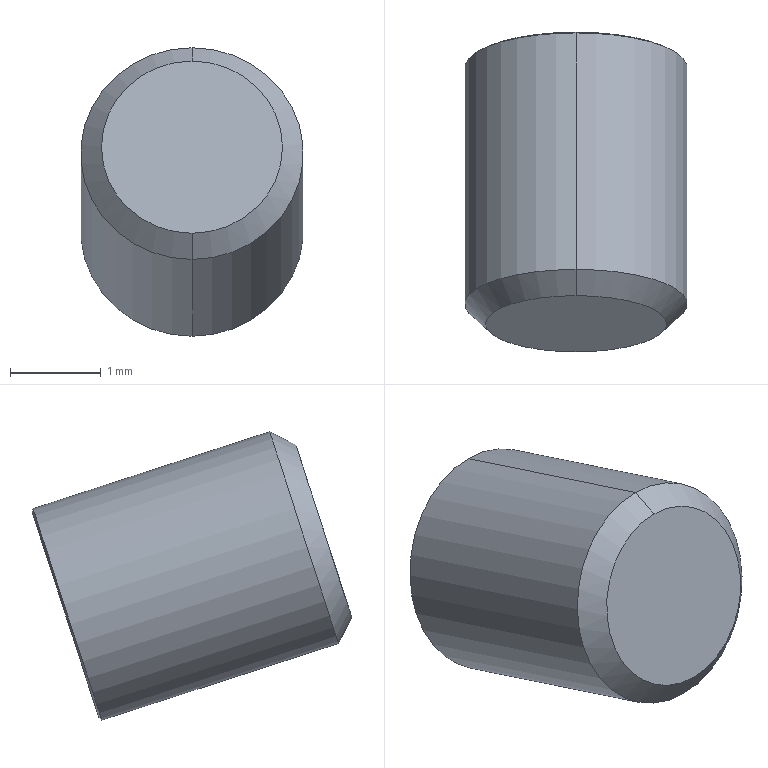Component | SolidWorks | Gewindestift_DIN_913_M3x3-1 | 1 solid | 22 faces | box 2.46 x 3.53 x 3.19 mm | volume 12 mm3 | cone 11 | plane 9 | cylinder 2 | commonest cylinder face diameters 2.459 x2
STEP:
#1=COLOUR_RGB('',0.7922,0.8196,0.9333);
#2=FILL_AREA_STYLE_COLOUR('',#1);
#3=FILL_AREA_STYLE('',(#2));
#4=SURFACE_STYLE_FILL_AREA(#3);
#5=SURFACE_SIDE_STYLE('',(#4));
#6=SURFACE_STYLE_USAGE(.BOTH.,#5);
#7=PRESENTATION_STYLE_ASSIGNMENT((#6));
#8=CARTESIAN_POINT('',(-0.5195,0.1896,-4.016));
#9=VERTEX_POINT('',#8);
#10=CARTESIAN_POINT('',(-0.5195,0.2186,-3.927));
#11=VERTEX_POINT('',#10);
#12=CARTESIAN_POINT('',(-0.5195,0.2041,-3.971));
#13=DIRECTION('',(0.,0.9512,-0.3087));
#14=DIRECTION('',(-0.,-0.3087,-0.9512));
#15=AXIS2_PLACEMENT_3D('',#12,#13,#14);
#16=CIRCLE('',#15,0.04699);
#17=EDGE_CURVE('',#9,#11,#16,.T.);
#18=ORIENTED_EDGE('',*,*,#17,.F.);
#19=CARTESIAN_POINT('',(-0.5195,0.1884,-4.017));
#20=VERTEX_POINT('',#19);
#21=CARTESIAN_POINT('',(-0.5195,0.1896,-4.016));
#22=DIRECTION('',(-0.,-0.7429,-0.6694));
#23=VECTOR('',#22,39.37);
#24=LINE('',#21,#23);
#25=EDGE_CURVE('',#9,#20,#24,.T.);
#26=ORIENTED_EDGE('',*,*,#25,.T.);
#27=CARTESIAN_POINT('',(-0.5195,0.2183,-3.925));
#28=VERTEX_POINT('',#27);
#29=CARTESIAN_POINT('',(-0.5195,0.2033,-3.971));
#30=DIRECTION('',(0.,0.9512,-0.3087));
#31=DIRECTION('',(-0.,0.3087,0.9512));
#32=AXIS2_PLACEMENT_3D('',#29,#30,#31);
#33=CIRCLE('',#32,0.04841);
#34=EDGE_CURVE('',#20,#28,#33,.T.);
#35=ORIENTED_EDGE('',*,*,#34,.T.);
#36=CARTESIAN_POINT('',(-0.5195,0.2186,-3.927));
#37=DIRECTION('',(0.,-0.2082,0.9781));
#38=VECTOR('',#37,39.37);
#39=LINE('',#36,#38);
#40=EDGE_CURVE('',#11,#28,#39,.T.);
#41=ORIENTED_EDGE('',*,*,#40,.F.);
#42=EDGE_LOOP('',(#18,#26,#35,#41));
#43=FACE_OUTER_BOUND('',#42,.T.);
#44=CARTESIAN_POINT('',(-0.5195,0.2041,-3.971));
#45=DIRECTION('',(-0.,-0.9512,0.3087));
#46=DIRECTION('',(0.,0.3087,0.9512));
#47=AXIS2_PLACEMENT_3D('',#44,#45,#46);
#48=CONICAL_SURFACE('',#47,0.04699,1.047);
#49=ADVANCED_FACE('',(#43),#48,.T.);
#50=CARTESIAN_POINT('',(-0.5195,0.08541,-3.984));
#51=VERTEX_POINT('',#50);
#52=CARTESIAN_POINT('',(-0.5195,0.1153,-3.892));
#53=VERTEX_POINT('',#52);
#54=CARTESIAN_POINT('',(-0.5195,0.1004,-3.938));
#55=DIRECTION('',(0.,0.9512,-0.3087));
#56=DIRECTION('',(-0.,-0.3087,-0.9512));
#57=AXIS2_PLACEMENT_3D('',#54,#55,#56);
#58=CIRCLE('',#57,0.04841);
#59=EDGE_CURVE('',#51,#53,#58,.T.);
#60=ORIENTED_EDGE('',*,*,#59,.T.);
#61=CARTESIAN_POINT('',(-0.5195,0.2003,-3.919));
#62=DIRECTION('',(0.,0.9512,-0.3087));
#63=VECTOR('',#62,39.37);
#64=LINE('',#61,#63);
#65=EDGE_CURVE('',#53,#28,#64,.T.);
#66=ORIENTED_EDGE('',*,*,#65,.T.);
#67=ORIENTED_EDGE('',*,*,#34,.F.);
#68=CARTESIAN_POINT('',(-0.5195,0.1704,-4.011));
#69=DIRECTION('',(0.,0.9512,-0.3087));
#70=VECTOR('',#69,39.37);
#71=LINE('',#68,#70);
#72=EDGE_CURVE('',#51,#20,#71,.T.);
#73=ORIENTED_EDGE('',*,*,#72,.F.);
#74=EDGE_LOOP('',(#60,#66,#67,#73));
#75=FACE_OUTER_BOUND('',#74,.T.);
#76=CARTESIAN_POINT('',(-0.5195,0.1854,-3.965));
#77=DIRECTION('',(0.,0.9512,-0.3087));
#78=DIRECTION('',(-0.,-0.3087,-0.9512));
#79=AXIS2_PLACEMENT_3D('',#76,#77,#78);
#80=CYLINDRICAL_SURFACE('',#79,0.04841);
#81=ADVANCED_FACE('',(#75),#80,.T.);
#82=CARTESIAN_POINT('',(-0.5195,0.07961,-3.972));
#83=VERTEX_POINT('',#82);
#84=CARTESIAN_POINT('',(-0.5195,0.1039,-3.897));
#85=VERTEX_POINT('',#84);
#86=CARTESIAN_POINT('',(-0.5195,0.09176,-3.935));
#87=DIRECTION('',(0.,0.9512,-0.3087));
#88=DIRECTION('',(-0.,-0.3087,-0.9512));
#89=AXIS2_PLACEMENT_3D('',#86,#87,#88);
#90=CIRCLE('',#89,0.03937);
#91=EDGE_CURVE('',#83,#85,#90,.T.);
#92=ORIENTED_EDGE('',*,*,#91,.T.);
#93=CARTESIAN_POINT('',(-0.5195,0.1287,-3.885));
#94=DIRECTION('',(0.,0.8909,0.4543));
#95=VECTOR('',#94,39.37);
#96=LINE('',#93,#95);
#97=EDGE_CURVE('',#85,#53,#96,.T.);
#98=ORIENTED_EDGE('',*,*,#97,.T.);
#99=ORIENTED_EDGE('',*,*,#59,.F.);
#100=CARTESIAN_POINT('',(-0.5195,0.09225,-3.997));
#101=DIRECTION('',(0.,0.4543,-0.8909));
#102=VECTOR('',#101,39.37);
#103=LINE('',#100,#102);
#104=EDGE_CURVE('',#83,#51,#103,.T.);
#105=ORIENTED_EDGE('',*,*,#104,.F.);
#106=EDGE_LOOP('',(#92,#98,#99,#105));
#107=FACE_OUTER_BOUND('',#106,.T.);
#108=CARTESIAN_POINT('',(-0.5195,0.1105,-3.941));
#109=DIRECTION('',(0.,0.9512,-0.3087));
#110=DIRECTION('',(-0.,-0.3087,-0.9512));
#111=AXIS2_PLACEMENT_3D('',#108,#109,#110);
#112=CONICAL_SURFACE('',#111,0.05906,0.7854);
#113=ADVANCED_FACE('',(#107),#112,.T.);
#114=CARTESIAN_POINT('',(-0.5365,0.195,-3.999));
#115=VERTEX_POINT('',#114);
#116=CARTESIAN_POINT('',(-0.5195,0.1925,-3.999));
#117=VERTEX_POINT('',#116);
#118=CARTESIAN_POINT('',(-0.5365,0.195,-3.999));
#119=CARTESIAN_POINT('',(-0.531,0.1935,-3.999));
#120=CARTESIAN_POINT('',(-0.5252,0.1925,-3.999));
#121=CARTESIAN_POINT('',(-0.5195,0.1925,-3.999));
#122=B_SPLINE_CURVE_WITH_KNOTS('',3,(#118,#119,#120,#121),.UNSPECIFIED.,.F.,.F.,(4,4),(0.002319,0.002758),.UNSPECIFIED.);
#123=EDGE_CURVE('',#115,#117,#122,.T.);
#124=ORIENTED_EDGE('',*,*,#123,.T.);
#125=CARTESIAN_POINT('',(-0.5195,0.1936,-4.004));
#126=VERTEX_POINT('',#125);
#127=CARTESIAN_POINT('',(-0.5195,0.1854,-3.965));
#128=DIRECTION('',(-0.,0.2082,-0.9781));
#129=VECTOR('',#128,39.37);
#130=LINE('',#127,#129);
#131=EDGE_CURVE('',#117,#126,#130,.T.);
#132=ORIENTED_EDGE('',*,*,#131,.T.);
#133=CARTESIAN_POINT('',(-0.5195,0.2041,-3.971));
#134=DIRECTION('',(0.,0.9512,-0.3087));
#135=DIRECTION('',(-0.,-0.3087,-0.9512));
#136=AXIS2_PLACEMENT_3D('',#133,#134,#135);
#137=CIRCLE('',#136,0.0341);
#138=EDGE_CURVE('',#126,#115,#137,.T.);
#139=ORIENTED_EDGE('',*,*,#138,.T.);
#140=EDGE_LOOP('',(#124,#132,#139));
#141=FACE_OUTER_BOUND('',#140,.T.);
#142=CARTESIAN_POINT('',(-0.5195,37.633,-16.119));
#143=DIRECTION('',(0.,0.9512,-0.3087));
#144=DIRECTION('',(-0.,-0.3087,-0.9512));
#145=AXIS2_PLACEMENT_3D('',#142,#143,#144);
#146=CONICAL_SURFACE('',#145,68.191,1.047);
#147=ADVANCED_FACE('',(#141),#146,.F.);
#148=CARTESIAN_POINT('',(-0.5536,0.2041,-3.971));
#149=VERTEX_POINT('',#148);
#150=CARTESIAN_POINT('',(-0.5365,0.2132,-3.943));
#151=VERTEX_POINT('',#150);
#152=CARTESIAN_POINT('',(-0.5195,0.2041,-3.971));
#153=DIRECTION('',(0.,0.9512,-0.3087));
#154=DIRECTION('',(-0.,-0.3087,-0.9512));
#155=AXIS2_PLACEMENT_3D('',#152,#153,#154);
#156=CIRCLE('',#155,0.0341);
#157=EDGE_CURVE('',#149,#151,#156,.T.);
#158=ORIENTED_EDGE('',*,*,#157,.T.);
#159=CARTESIAN_POINT('',(-0.5365,0.2132,-3.943));
#160=CARTESIAN_POINT('',(-0.5393,0.2102,-3.947));
#161=CARTESIAN_POINT('',(-0.5421,0.2077,-3.952));
#162=CARTESIAN_POINT('',(-0.5479,0.2046,-3.961));
#163=CARTESIAN_POINT('',(-0.5508,0.2041,-3.966));
#164=CARTESIAN_POINT('',(-0.5536,0.2041,-3.971));
#165=B_SPLINE_CURVE_WITH_KNOTS('',3,(#159,#160,#161,#162,#163,#164),.UNSPECIFIED.,.F.,.F.,(4,2,4),(0.00000024,0.0004376,0.0008749),.UNSPECIFIED.);
#166=EDGE_CURVE('',#151,#149,#165,.T.);
#167=ORIENTED_EDGE('',*,*,#166,.T.);
#168=EDGE_LOOP('',(#158,#167));
#169=FACE_OUTER_BOUND('',#168,.T.);
#170=CARTESIAN_POINT('',(-0.5195,37.633,-16.119));
#171=DIRECTION('',(0.,0.9512,-0.3087));
#172=DIRECTION('',(-0.,-0.3087,-0.9512));
#173=AXIS2_PLACEMENT_3D('',#170,#171,#172);
#174=CONICAL_SURFACE('',#173,68.191,1.047);
#175=ADVANCED_FACE('',(#169),#174,.F.);
#176=CARTESIAN_POINT('',(-0.5195,0.2041,-3.971));
#177=DIRECTION('',(0.,0.9512,-0.3087));
#178=DIRECTION('',(-0.,-0.3087,-0.9512));
#179=AXIS2_PLACEMENT_3D('',#176,#177,#178);
#180=CIRCLE('',#179,0.0341);
#181=EDGE_CURVE('',#115,#149,#180,.T.);
#182=ORIENTED_EDGE('',*,*,#181,.T.);
#183=CARTESIAN_POINT('',(-0.5536,0.2041,-3.971));
#184=CARTESIAN_POINT('',(-0.5508,0.2011,-3.975));
#185=CARTESIAN_POINT('',(-0.548,0.1986,-3.98));
#186=CARTESIAN_POINT('',(-0.5422,0.1955,-3.989));
#187=CARTESIAN_POINT('',(-0.5393,0.1949,-3.994));
#188=CARTESIAN_POINT('',(-0.5365,0.195,-3.999));
#189=B_SPLINE_CURVE_WITH_KNOTS('',3,(#183,#184,#185,#186,#187,#188),.UNSPECIFIED.,.F.,.F.,(4,2,4),(0.00000024,0.0004376,0.0008749),.UNSPECIFIED.);
#190=EDGE_CURVE('',#149,#115,#189,.T.);
#191=ORIENTED_EDGE('',*,*,#190,.T.);
#192=EDGE_LOOP('',(#182,#191));
#193=FACE_OUTER_BOUND('',#192,.T.);
#194=CARTESIAN_POINT('',(-0.5195,37.633,-16.119));
#195=DIRECTION('',(0.,0.9512,-0.3087));
#196=DIRECTION('',(-0.,-0.3087,-0.9512));
#197=AXIS2_PLACEMENT_3D('',#194,#195,#196);
#198=CONICAL_SURFACE('',#197,68.191,1.047);
#199=ADVANCED_FACE('',(#193),#198,.F.);
#200=ORIENTED_EDGE('',*,*,#131,.F.);
#201=CARTESIAN_POINT('',(-0.5024,0.195,-3.999));
#202=VERTEX_POINT('',#201);
#203=CARTESIAN_POINT('',(-0.5195,0.1925,-3.999));
#204=CARTESIAN_POINT('',(-0.5137,0.1925,-3.999));
#205=CARTESIAN_POINT('',(-0.508,0.1935,-3.999));
#206=CARTESIAN_POINT('',(-0.5024,0.195,-3.999));
#207=B_SPLINE_CURVE_WITH_KNOTS('',3,(#203,#204,#205,#206),.UNSPECIFIED.,.F.,.F.,(4,4),(0.002758,0.003196),.UNSPECIFIED.);
#208=EDGE_CURVE('',#117,#202,#207,.T.);
#209=ORIENTED_EDGE('',*,*,#208,.T.);
#210=CARTESIAN_POINT('',(-0.5195,0.2041,-3.971));
#211=DIRECTION('',(0.,0.9512,-0.3087));
#212=DIRECTION('',(-0.,-0.3087,-0.9512));
#213=AXIS2_PLACEMENT_3D('',#210,#211,#212);
#214=CIRCLE('',#213,0.0341);
#215=EDGE_CURVE('',#202,#126,#214,.T.);
#216=ORIENTED_EDGE('',*,*,#215,.T.);
#217=EDGE_LOOP('',(#200,#209,#216));
#218=FACE_OUTER_BOUND('',#217,.T.);
#219=CARTESIAN_POINT('',(-0.5195,37.633,-16.119));
#220=DIRECTION('',(0.,0.9512,-0.3087));
#221=DIRECTION('',(-0.,-0.3087,-0.9512));
#222=AXIS2_PLACEMENT_3D('',#219,#220,#221);
#223=CONICAL_SURFACE('',#222,68.191,1.047);
#224=ADVANCED_FACE('',(#218),#223,.F.);
#225=CARTESIAN_POINT('',(-0.4854,0.2041,-3.971));
#226=VERTEX_POINT('',#225);
#227=CARTESIAN_POINT('',(-0.5195,0.2041,-3.971));
#228=DIRECTION('',(0.,0.9512,-0.3087));
#229=DIRECTION('',(-0.,-0.3087,-0.9512));
#230=AXIS2_PLACEMENT_3D('',#227,#228,#229);
#231=CIRCLE('',#230,0.0341);
#232=EDGE_CURVE('',#226,#202,#231,.T.);
#233=ORIENTED_EDGE('',*,*,#232,.T.);
#234=CARTESIAN_POINT('',(-0.5024,0.195,-3.999));
#235=CARTESIAN_POINT('',(-0.4996,0.1949,-3.994));
#236=CARTESIAN_POINT('',(-0.4968,0.1955,-3.989));
#237=CARTESIAN_POINT('',(-0.491,0.1986,-3.98));
#238=CARTESIAN_POINT('',(-0.4882,0.2011,-3.975));
#239=CARTESIAN_POINT('',(-0.4854,0.2041,-3.971));
#240=B_SPLINE_CURVE_WITH_KNOTS('',3,(#234,#235,#236,#237,#238,#239),.UNSPECIFIED.,.F.,.F.,(4,2,4),(0.00000024,0.0004376,0.0008749),.UNSPECIFIED.);
#241=EDGE_CURVE('',#202,#226,#240,.T.);
#242=ORIENTED_EDGE('',*,*,#241,.T.);
#243=EDGE_LOOP('',(#233,#242));
#244=FACE_OUTER_BOUND('',#243,.T.);
#245=CARTESIAN_POINT('',(-0.5195,37.633,-16.119));
#246=DIRECTION('',(0.,0.9512,-0.3087));
#247=DIRECTION('',(-0.,-0.3087,-0.9512));
#248=AXIS2_PLACEMENT_3D('',#245,#246,#247);
#249=CONICAL_SURFACE('',#248,68.191,1.047);
#250=ADVANCED_FACE('',(#244),#249,.F.);
#251=CARTESIAN_POINT('',(-0.5024,0.2132,-3.943));
#252=VERTEX_POINT('',#251);
#253=CARTESIAN_POINT('',(-0.5195,0.2041,-3.971));
#254=DIRECTION('',(0.,0.9512,-0.3087));
#255=DIRECTION('',(-0.,-0.3087,-0.9512));
#256=AXIS2_PLACEMENT_3D('',#253,#254,#255);
#257=CIRCLE('',#256,0.0341);
#258=EDGE_CURVE('',#252,#226,#257,.T.);
#259=ORIENTED_EDGE('',*,*,#258,.T.);
#260=CARTESIAN_POINT('',(-0.4854,0.2041,-3.971));
#261=CARTESIAN_POINT('',(-0.4882,0.2041,-3.966));
#262=CARTESIAN_POINT('',(-0.491,0.2046,-3.961));
#263=CARTESIAN_POINT('',(-0.4968,0.2077,-3.952));
#264=CARTESIAN_POINT('',(-0.4996,0.2102,-3.947));
#265=CARTESIAN_POINT('',(-0.5024,0.2132,-3.943));
#266=B_SPLINE_CURVE_WITH_KNOTS('',3,(#260,#261,#262,#263,#264,#265),.UNSPECIFIED.,.F.,.F.,(4,2,4),(0.00000024,0.0004376,0.0008749),.UNSPECIFIED.);
#267=EDGE_CURVE('',#226,#252,#266,.T.);
#268=ORIENTED_EDGE('',*,*,#267,.T.);
#269=EDGE_LOOP('',(#259,#268));
#270=FACE_OUTER_BOUND('',#269,.T.);
#271=CARTESIAN_POINT('',(-0.5195,37.633,-16.119));
#272=DIRECTION('',(0.,0.9512,-0.3087));
#273=DIRECTION('',(-0.,-0.3087,-0.9512));
#274=AXIS2_PLACEMENT_3D('',#271,#272,#273);
#275=CONICAL_SURFACE('',#274,68.191,1.047);
#276=ADVANCED_FACE('',(#270),#275,.F.);
#277=CARTESIAN_POINT('',(-0.5195,0.2041,-3.971));
#278=DIRECTION('',(0.,0.9512,-0.3087));
#279=DIRECTION('',(-0.,-0.3087,-0.9512));
#280=AXIS2_PLACEMENT_3D('',#277,#278,#279);
#281=CIRCLE('',#280,0.0341);
#282=EDGE_CURVE('',#151,#252,#281,.T.);
#283=ORIENTED_EDGE('',*,*,#282,.T.);
#284=CARTESIAN_POINT('',(-0.5024,0.2132,-3.943));
#285=CARTESIAN_POINT('',(-0.508,0.2117,-3.943));
#286=CARTESIAN_POINT('',(-0.5137,0.2107,-3.942));
#287=CARTESIAN_POINT('',(-0.5252,0.2107,-3.942));
#288=CARTESIAN_POINT('',(-0.531,0.2117,-3.943));
#289=CARTESIAN_POINT('',(-0.5365,0.2132,-3.943));
#290=B_SPLINE_CURVE_WITH_KNOTS('',3,(#284,#285,#286,#287,#288,#289),.UNSPECIFIED.,.F.,.F.,(4,2,4),(0.0007425,0.00118,0.001618),.UNSPECIFIED.);
#291=EDGE_CURVE('',#252,#151,#290,.T.);
#292=ORIENTED_EDGE('',*,*,#291,.T.);
#293=EDGE_LOOP('',(#283,#292));
#294=FACE_OUTER_BOUND('',#293,.T.);
#295=CARTESIAN_POINT('',(-0.5195,37.633,-16.119));
#296=DIRECTION('',(0.,0.9512,-0.3087));
#297=DIRECTION('',(-0.,-0.3087,-0.9512));
#298=AXIS2_PLACEMENT_3D('',#295,#296,#297);
#299=CONICAL_SURFACE('',#298,68.191,1.047);
#300=ADVANCED_FACE('',(#294),#299,.F.);
#301=ORIENTED_EDGE('',*,*,#91,.F.);
#302=CARTESIAN_POINT('',(-0.5195,0.09176,-3.935));
#303=DIRECTION('',(0.,0.9512,-0.3087));
#304=DIRECTION('',(-0.,-0.3087,-0.9512));
#305=AXIS2_PLACEMENT_3D('',#302,#303,#304);
#306=CIRCLE('',#305,0.03937);
#307=EDGE_CURVE('',#85,#83,#306,.T.);
#308=ORIENTED_EDGE('',*,*,#307,.F.);
#309=EDGE_LOOP('',(#301,#308));
#310=FACE_OUTER_BOUND('',#309,.T.);
#311=CARTESIAN_POINT('',(-0.5195,0.09176,-3.935));
#312=DIRECTION('',(-0.,-0.9512,0.3087));
#313=DIRECTION('',(0.,0.3087,0.9512));
#314=AXIS2_PLACEMENT_3D('',#311,#312,#313);
#315=PLANE('',#314);
#316=ADVANCED_FACE('',(#310),#315,.T.);
#317=ORIENTED_EDGE('',*,*,#97,.F.);
#318=ORIENTED_EDGE('',*,*,#307,.T.);
#319=ORIENTED_EDGE('',*,*,#104,.T.);
#320=CARTESIAN_POINT('',(-0.5195,0.1004,-3.938));
#321=DIRECTION('',(0.,0.9512,-0.3087));
#322=DIRECTION('',(-0.,-0.3087,-0.9512));
#323=AXIS2_PLACEMENT_3D('',#320,#321,#322);
#324=CIRCLE('',#323,0.04841);
#325=EDGE_CURVE('',#53,#51,#324,.T.);
#326=ORIENTED_EDGE('',*,*,#325,.F.);
#327=EDGE_LOOP('',(#317,#318,#319,#326));
#328=FACE_OUTER_BOUND('',#327,.T.);
#329=CARTESIAN_POINT('',(-0.5195,0.1105,-3.941));
#330=DIRECTION('',(0.,0.9512,-0.3087));
#331=DIRECTION('',(-0.,-0.3087,-0.9512));
#332=AXIS2_PLACEMENT_3D('',#329,#330,#331);
#333=CONICAL_SURFACE('',#332,0.05906,0.7854);
#334=ADVANCED_FACE('',(#328),#333,.T.);
#335=ORIENTED_EDGE('',*,*,#65,.F.);
#336=ORIENTED_EDGE('',*,*,#325,.T.);
#337=ORIENTED_EDGE('',*,*,#72,.T.);
#338=CARTESIAN_POINT('',(-0.5195,0.2033,-3.971));
#339=DIRECTION('',(0.,0.9512,-0.3087));
#340=DIRECTION('',(0.,0.3087,0.9512));
#341=AXIS2_PLACEMENT_3D('',#338,#339,#340);
#342=CIRCLE('',#341,0.04841);
#343=EDGE_CURVE('',#28,#20,#342,.T.);
#344=ORIENTED_EDGE('',*,*,#343,.F.);
#345=EDGE_LOOP('',(#335,#336,#337,#344));
#346=FACE_OUTER_BOUND('',#345,.T.);
#347=CARTESIAN_POINT('',(-0.5195,0.1854,-3.965));
#348=DIRECTION('',(0.,0.9512,-0.3087));
#349=DIRECTION('',(-0.,-0.3087,-0.9512));
#350=AXIS2_PLACEMENT_3D('',#347,#348,#349);
#351=CYLINDRICAL_SURFACE('',#350,0.04841);
#352=ADVANCED_FACE('',(#346),#351,.T.);
#353=ORIENTED_EDGE('',*,*,#25,.F.);
#354=CARTESIAN_POINT('',(-0.5195,0.2041,-3.971));
#355=DIRECTION('',(0.,0.9512,-0.3087));
#356=DIRECTION('',(-0.,-0.3087,-0.9512));
#357=AXIS2_PLACEMENT_3D('',#354,#355,#356);
#358=CIRCLE('',#357,0.04699);
#359=EDGE_CURVE('',#11,#9,#358,.T.);
#360=ORIENTED_EDGE('',*,*,#359,.F.);
#361=ORIENTED_EDGE('',*,*,#40,.T.);
#362=ORIENTED_EDGE('',*,*,#343,.T.);
#363=EDGE_LOOP('',(#353,#360,#361,#362));
#364=FACE_OUTER_BOUND('',#363,.T.);
#365=CARTESIAN_POINT('',(-0.5195,0.2041,-3.971));
#366=DIRECTION('',(-0.,-0.9512,0.3087));
#367=DIRECTION('',(0.,0.3087,0.9512));
#368=AXIS2_PLACEMENT_3D('',#365,#366,#367);
#369=CONICAL_SURFACE('',#368,0.04699,1.047);
#370=ADVANCED_FACE('',(#364),#369,.T.);
#371=ORIENTED_EDGE('',*,*,#359,.T.);
#372=ORIENTED_EDGE('',*,*,#17,.T.);
#373=EDGE_LOOP('',(#371,#372));
#374=FACE_OUTER_BOUND('',#373,.T.);
#375=ORIENTED_EDGE('',*,*,#181,.F.);
#376=ORIENTED_EDGE('',*,*,#138,.F.);
#377=ORIENTED_EDGE('',*,*,#215,.F.);
#378=ORIENTED_EDGE('',*,*,#232,.F.);
#379=ORIENTED_EDGE('',*,*,#258,.F.);
#380=ORIENTED_EDGE('',*,*,#282,.F.);
#381=ORIENTED_EDGE('',*,*,#157,.F.);
#382=EDGE_LOOP('',(#375,#376,#377,#378,#379,#380,#381));
#383=FACE_BOUND('',#382,.T.);
#384=CARTESIAN_POINT('',(-0.5195,0.1896,-4.016));
#385=DIRECTION('',(0.,0.9512,-0.3087));
#386=DIRECTION('',(-0.,-0.3087,-0.9512));
#387=AXIS2_PLACEMENT_3D('',#384,#385,#386);
#388=PLANE('',#387);
#389=ADVANCED_FACE('',(#374,#383),#388,.T.);
#390=CARTESIAN_POINT('',(-0.5365,0.1683,-3.929));
#391=VERTEX_POINT('',#390);
#392=CARTESIAN_POINT('',(-0.5365,0.1683,-3.929));
#393=DIRECTION('',(0.,0.9512,-0.3087));
#394=VECTOR('',#393,39.37);
#395=LINE('',#392,#394);
#396=EDGE_CURVE('',#391,#151,#395,.T.);
#397=ORIENTED_EDGE('',*,*,#396,.F.);
#398=CARTESIAN_POINT('',(-0.5536,0.1592,-3.957));
#399=VERTEX_POINT('',#398);
#400=CARTESIAN_POINT('',(-0.5365,0.1683,-3.929));
#401=DIRECTION('',(-0.5,-0.2673,-0.8237));
#402=VECTOR('',#401,39.37);
#403=LINE('',#400,#402);
#404=EDGE_CURVE('',#391,#399,#403,.T.);
#405=ORIENTED_EDGE('',*,*,#404,.T.);
#406=CARTESIAN_POINT('',(-0.5536,0.1592,-3.957));
#407=DIRECTION('',(0.,0.9512,-0.3087));
#408=VECTOR('',#407,39.37);
#409=LINE('',#406,#408);
#410=EDGE_CURVE('',#399,#149,#409,.T.);
#411=ORIENTED_EDGE('',*,*,#410,.T.);
#412=ORIENTED_EDGE('',*,*,#166,.F.);
#413=EDGE_LOOP('',(#397,#405,#411,#412));
#414=FACE_OUTER_BOUND('',#413,.T.);
#415=CARTESIAN_POINT('',(-0.5365,0.1683,-3.929));
#416=DIRECTION('',(0.866,-0.1544,-0.4756));
#417=DIRECTION('',(0.5,0.2673,0.8237));
#418=AXIS2_PLACEMENT_3D('',#415,#416,#417);
#419=PLANE('',#418);
#420=ADVANCED_FACE('',(#414),#419,.T.);
#421=ORIENTED_EDGE('',*,*,#410,.F.);
#422=CARTESIAN_POINT('',(-0.5365,0.1501,-3.985));
#423=VERTEX_POINT('',#422);
#424=CARTESIAN_POINT('',(-0.5536,0.1592,-3.957));
#425=DIRECTION('',(0.5,-0.2673,-0.8237));
#426=VECTOR('',#425,39.37);
#427=LINE('',#424,#426);
#428=EDGE_CURVE('',#399,#423,#427,.T.);
#429=ORIENTED_EDGE('',*,*,#428,.T.);
#430=CARTESIAN_POINT('',(-0.5365,0.1501,-3.985));
#431=DIRECTION('',(0.,0.9512,-0.3087));
#432=VECTOR('',#431,39.37);
#433=LINE('',#430,#432);
#434=EDGE_CURVE('',#423,#115,#433,.T.);
#435=ORIENTED_EDGE('',*,*,#434,.T.);
#436=ORIENTED_EDGE('',*,*,#190,.F.);
#437=EDGE_LOOP('',(#421,#429,#435,#436));
#438=FACE_OUTER_BOUND('',#437,.T.);
#439=CARTESIAN_POINT('',(-0.5536,0.1592,-3.957));
#440=DIRECTION('',(0.866,0.1544,0.4756));
#441=DIRECTION('',(-0.5,0.2673,0.8237));
#442=AXIS2_PLACEMENT_3D('',#439,#440,#441);
#443=PLANE('',#442);
#444=ADVANCED_FACE('',(#438),#443,.T.);
#445=ORIENTED_EDGE('',*,*,#434,.F.);
#446=CARTESIAN_POINT('',(-0.5024,0.1501,-3.985));
#447=VERTEX_POINT('',#446);
#448=CARTESIAN_POINT('',(-0.5365,0.1501,-3.985));
#449=DIRECTION('',(1.,-0.,0.));
#450=VECTOR('',#449,39.37);
#451=LINE('',#448,#450);
#452=EDGE_CURVE('',#423,#447,#451,.T.);
#453=ORIENTED_EDGE('',*,*,#452,.T.);
#454=CARTESIAN_POINT('',(-0.5024,0.1501,-3.985));
#455=DIRECTION('',(0.,0.9512,-0.3087));
#456=VECTOR('',#455,39.37);
#457=LINE('',#454,#456);
#458=EDGE_CURVE('',#447,#202,#457,.T.);
#459=ORIENTED_EDGE('',*,*,#458,.T.);
#460=ORIENTED_EDGE('',*,*,#208,.F.);
#461=ORIENTED_EDGE('',*,*,#123,.F.);
#462=EDGE_LOOP('',(#445,#453,#459,#460,#461));
#463=FACE_OUTER_BOUND('',#462,.T.);
#464=CARTESIAN_POINT('',(-0.5365,0.1501,-3.985));
#465=DIRECTION('',(0.,0.3087,0.9512));
#466=DIRECTION('',(-1.,0.,-0.));
#467=AXIS2_PLACEMENT_3D('',#464,#465,#466);
#468=PLANE('',#467);
#469=ADVANCED_FACE('',(#463),#468,.T.);
#470=ORIENTED_EDGE('',*,*,#458,.F.);
#471=CARTESIAN_POINT('',(-0.4854,0.1592,-3.957));
#472=VERTEX_POINT('',#471);
#473=CARTESIAN_POINT('',(-0.5024,0.1501,-3.985));
#474=DIRECTION('',(0.5,0.2673,0.8237));
#475=VECTOR('',#474,39.37);
#476=LINE('',#473,#475);
#477=EDGE_CURVE('',#447,#472,#476,.T.);
#478=ORIENTED_EDGE('',*,*,#477,.T.);
#479=CARTESIAN_POINT('',(-0.4854,0.1592,-3.957));
#480=DIRECTION('',(0.,0.9512,-0.3087));
#481=VECTOR('',#480,39.37);
#482=LINE('',#479,#481);
#483=EDGE_CURVE('',#472,#226,#482,.T.);
#484=ORIENTED_EDGE('',*,*,#483,.T.);
#485=ORIENTED_EDGE('',*,*,#241,.F.);
#486=EDGE_LOOP('',(#470,#478,#484,#485));
#487=FACE_OUTER_BOUND('',#486,.T.);
#488=CARTESIAN_POINT('',(-0.5024,0.1501,-3.985));
#489=DIRECTION('',(-0.866,0.1544,0.4756));
#490=DIRECTION('',(-0.5,-0.2673,-0.8237));
#491=AXIS2_PLACEMENT_3D('',#488,#489,#490);
#492=PLANE('',#491);
#493=ADVANCED_FACE('',(#487),#492,.T.);
#494=ORIENTED_EDGE('',*,*,#483,.F.);
#495=CARTESIAN_POINT('',(-0.5024,0.1683,-3.929));
#496=VERTEX_POINT('',#495);
#497=CARTESIAN_POINT('',(-0.4854,0.1592,-3.957));
#498=DIRECTION('',(-0.5,0.2673,0.8237));
#499=VECTOR('',#498,39.37);
#500=LINE('',#497,#499);
#501=EDGE_CURVE('',#472,#496,#500,.T.);
#502=ORIENTED_EDGE('',*,*,#501,.T.);
#503=CARTESIAN_POINT('',(-0.5024,0.1683,-3.929));
#504=DIRECTION('',(0.,0.9512,-0.3087));
#505=VECTOR('',#504,39.37);
#506=LINE('',#503,#505);
#507=EDGE_CURVE('',#496,#252,#506,.T.);
#508=ORIENTED_EDGE('',*,*,#507,.T.);
#509=ORIENTED_EDGE('',*,*,#267,.F.);
#510=EDGE_LOOP('',(#494,#502,#508,#509));
#511=FACE_OUTER_BOUND('',#510,.T.);
#512=CARTESIAN_POINT('',(-0.4854,0.1592,-3.957));
#513=DIRECTION('',(-0.866,-0.1544,-0.4756));
#514=DIRECTION('',(0.5,-0.2673,-0.8237));
#515=AXIS2_PLACEMENT_3D('',#512,#513,#514);
#516=PLANE('',#515);
#517=ADVANCED_FACE('',(#511),#516,.T.);
#518=ORIENTED_EDGE('',*,*,#507,.F.);
#519=CARTESIAN_POINT('',(-0.5024,0.1683,-3.929));
#520=DIRECTION('',(-1.,0.,-0.));
#521=VECTOR('',#520,39.37);
#522=LINE('',#519,#521);
#523=EDGE_CURVE('',#496,#391,#522,.T.);
#524=ORIENTED_EDGE('',*,*,#523,.T.);
#525=ORIENTED_EDGE('',*,*,#396,.T.);
#526=ORIENTED_EDGE('',*,*,#291,.F.);
#527=EDGE_LOOP('',(#518,#524,#525,#526));
#528=FACE_OUTER_BOUND('',#527,.T.);
#529=CARTESIAN_POINT('',(-0.5024,0.1683,-3.929));
#530=DIRECTION('',(-0.,-0.3087,-0.9512));
#531=DIRECTION('',(1.,-0.,0.));
#532=AXIS2_PLACEMENT_3D('',#529,#530,#531);
#533=PLANE('',#532);
#534=ADVANCED_FACE('',(#528),#533,.T.);
#535=ORIENTED_EDGE('',*,*,#404,.F.);
#536=ORIENTED_EDGE('',*,*,#523,.F.);
#537=ORIENTED_EDGE('',*,*,#501,.F.);
#538=ORIENTED_EDGE('',*,*,#477,.F.);
#539=ORIENTED_EDGE('',*,*,#452,.F.);
#540=ORIENTED_EDGE('',*,*,#428,.F.);
#541=EDGE_LOOP('',(#535,#536,#537,#538,#539,#540));
#542=FACE_OUTER_BOUND('',#541,.T.);
#543=CARTESIAN_POINT('',(-0.5195,0.1592,-3.957));
#544=DIRECTION('',(-0.,-0.9512,0.3087));
#545=DIRECTION('',(1.,-0.,0.));
#546=AXIS2_PLACEMENT_3D('',#543,#544,#545);
#547=PLANE('',#546);
#548=ADVANCED_FACE('',(#542),#547,.F.);
#549=CLOSED_SHELL('',(#49,#81,#113,#147,#175,#199,#224,#250,#276,#300,#316,#334,#352,#370,#389,#420,#444,#469,#493,#517,#534,#548));
#550=MANIFOLD_SOLID_BREP('',#549);
#551=STYLED_ITEM('',(#7),#550);
#552=PRESENTATION_LAYER_ASSIGNMENT('','',(#551));
#553=(LENGTH_UNIT()NAMED_UNIT(*)SI_UNIT($,.METRE.));
#554=LENGTH_MEASURE_WITH_UNIT(LENGTH_MEASURE(0.0254),#553);
#555=DIMENSIONAL_EXPONENTS(1.,0.,0.,0.,0.,0.,0.);
#556=(CONVERSION_BASED_UNIT('',#554)LENGTH_UNIT()NAMED_UNIT(#555));
#557=UNCERTAINTY_MEASURE_WITH_UNIT(LENGTH_MEASURE(0.00001),#556,'','');
#558=(NAMED_UNIT(*)PLANE_ANGLE_UNIT()SI_UNIT($,.RADIAN.));
#559=(NAMED_UNIT(*)SI_UNIT($,.STERADIAN.)SOLID_ANGLE_UNIT());
#560=(GEOMETRIC_REPRESENTATION_CONTEXT(3)GLOBAL_UNCERTAINTY_ASSIGNED_CONTEXT((#557))GLOBAL_UNIT_ASSIGNED_CONTEXT((#556,#558,#559))REPRESENTATION_CONTEXT('',''));
#561=MECHANICAL_DESIGN_GEOMETRIC_PRESENTATION_REPRESENTATION('',(#551),#560);
#562=CARTESIAN_POINT('',(0.,0.,0.));
#563=DIRECTION('',(0.,0.,1.));
#564=DIRECTION('',(1.,0.,0.));
#565=AXIS2_PLACEMENT_3D('',#562,#563,#564);
#566=(LENGTH_UNIT()NAMED_UNIT(*)SI_UNIT($,.METRE.));
#567=LENGTH_MEASURE_WITH_UNIT(LENGTH_MEASURE(0.0254),#566);
#568=DIMENSIONAL_EXPONENTS(1.,0.,0.,0.,0.,0.,0.);
#569=(CONVERSION_BASED_UNIT('',#567)LENGTH_UNIT()NAMED_UNIT(#568));
#570=UNCERTAINTY_MEASURE_WITH_UNIT(LENGTH_MEASURE(0.00001),#569,'','');
#571=(NAMED_UNIT(*)PLANE_ANGLE_UNIT()SI_UNIT($,.RADIAN.));
#572=(NAMED_UNIT(*)SI_UNIT($,.STERADIAN.)SOLID_ANGLE_UNIT());
#573=(GEOMETRIC_REPRESENTATION_CONTEXT(3)GLOBAL_UNCERTAINTY_ASSIGNED_CONTEXT((#570))GLOBAL_UNIT_ASSIGNED_CONTEXT((#569,#571,#572))REPRESENTATION_CONTEXT('',''));
#574=ADVANCED_BREP_SHAPE_REPRESENTATION('',(#550,#565),#573);